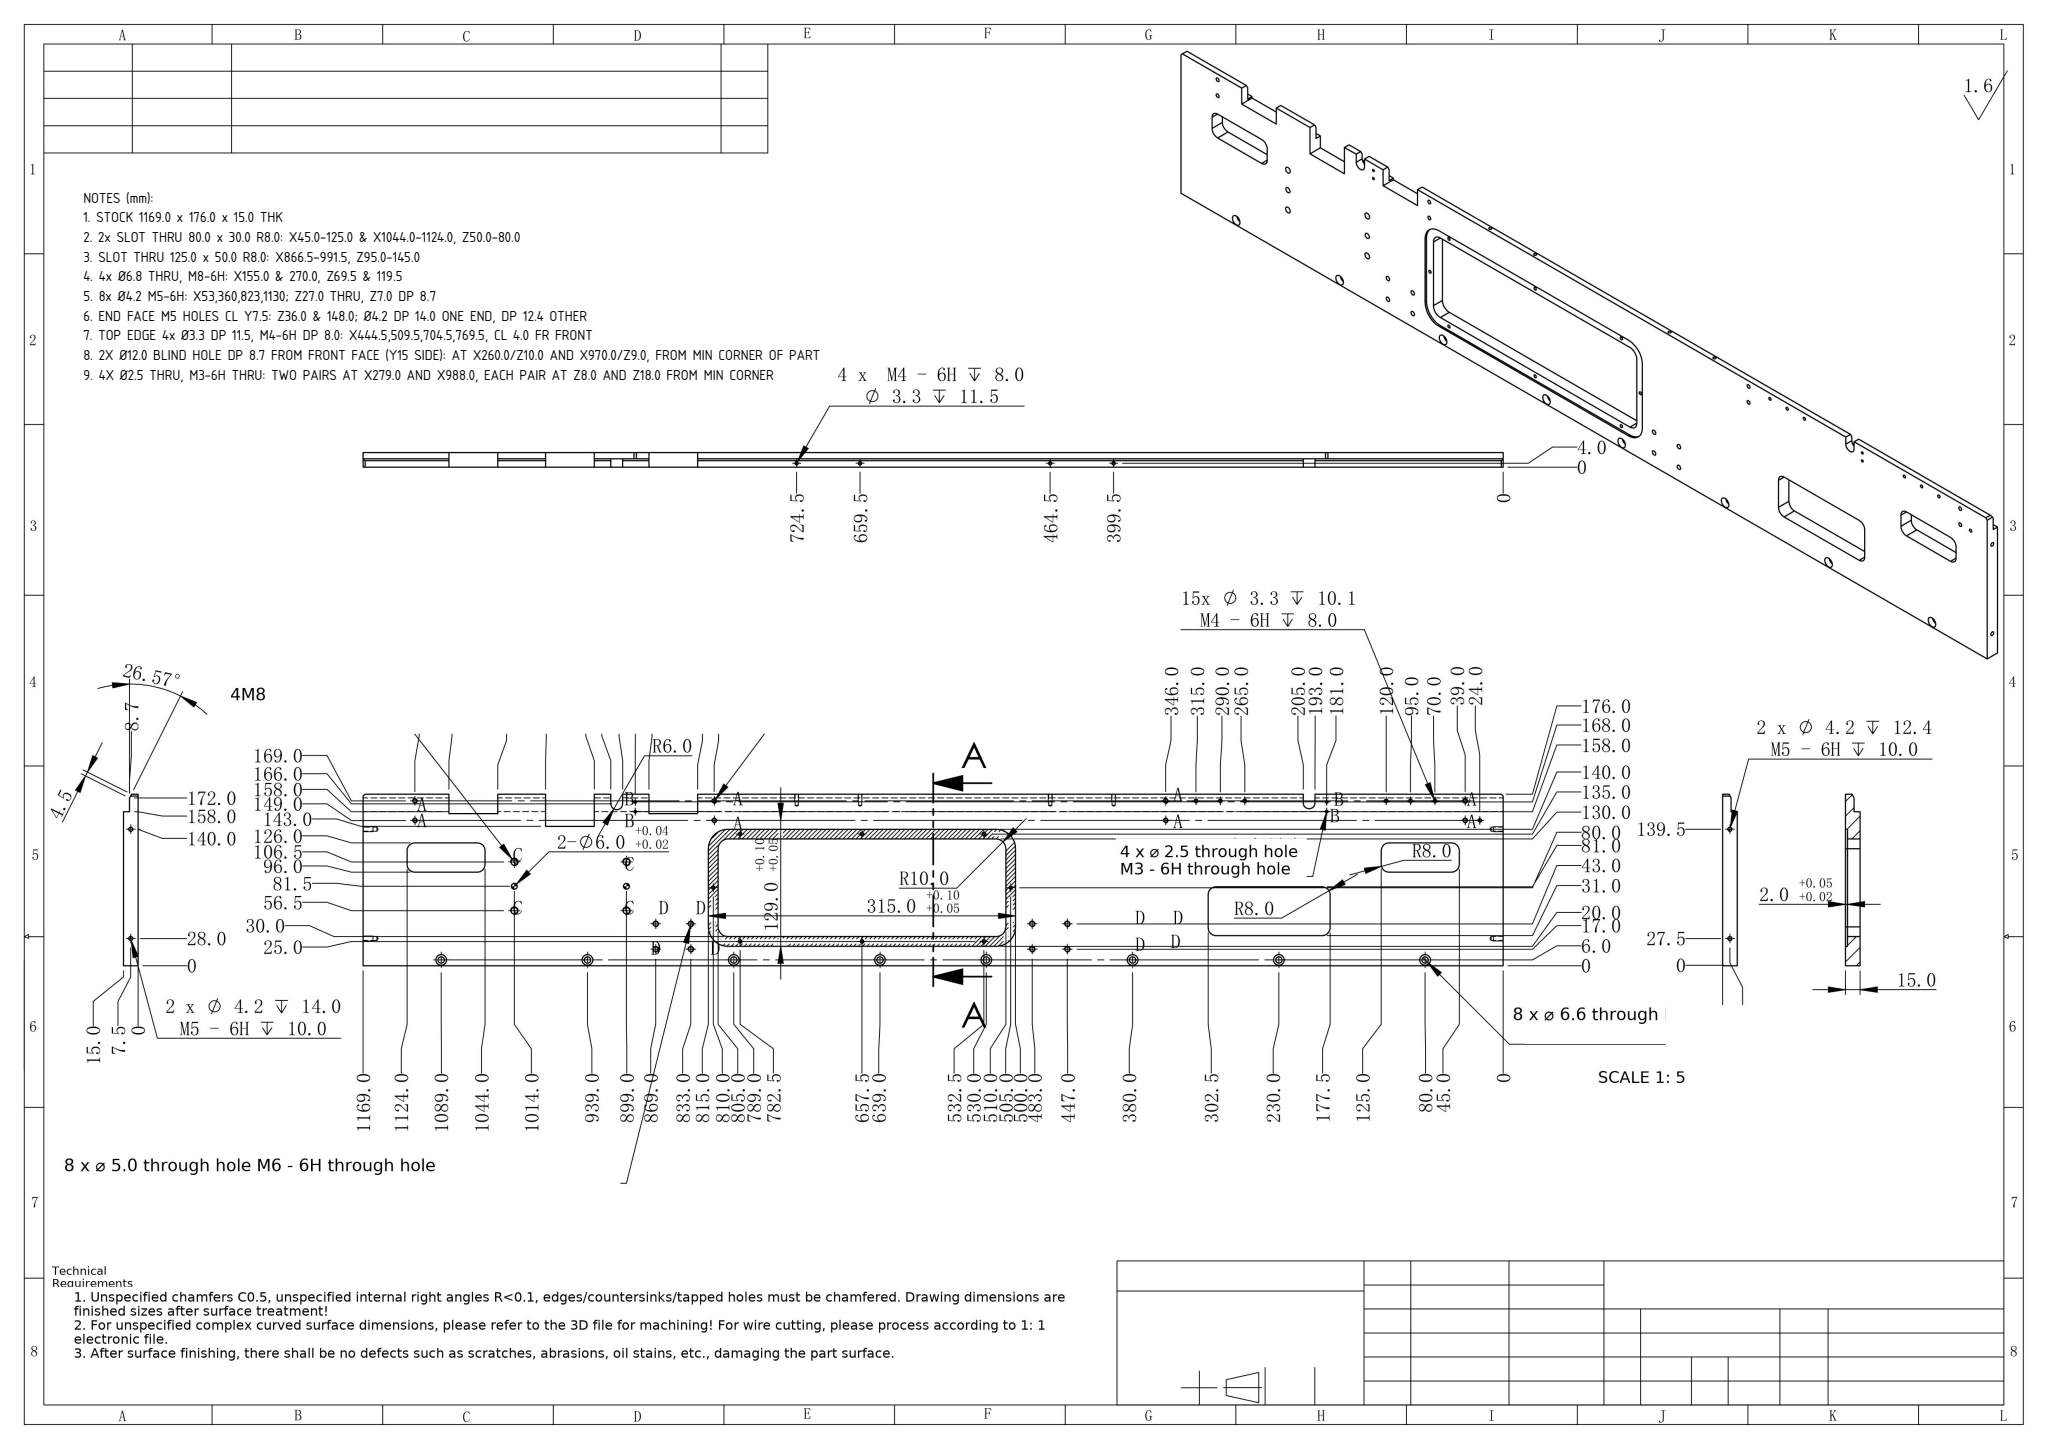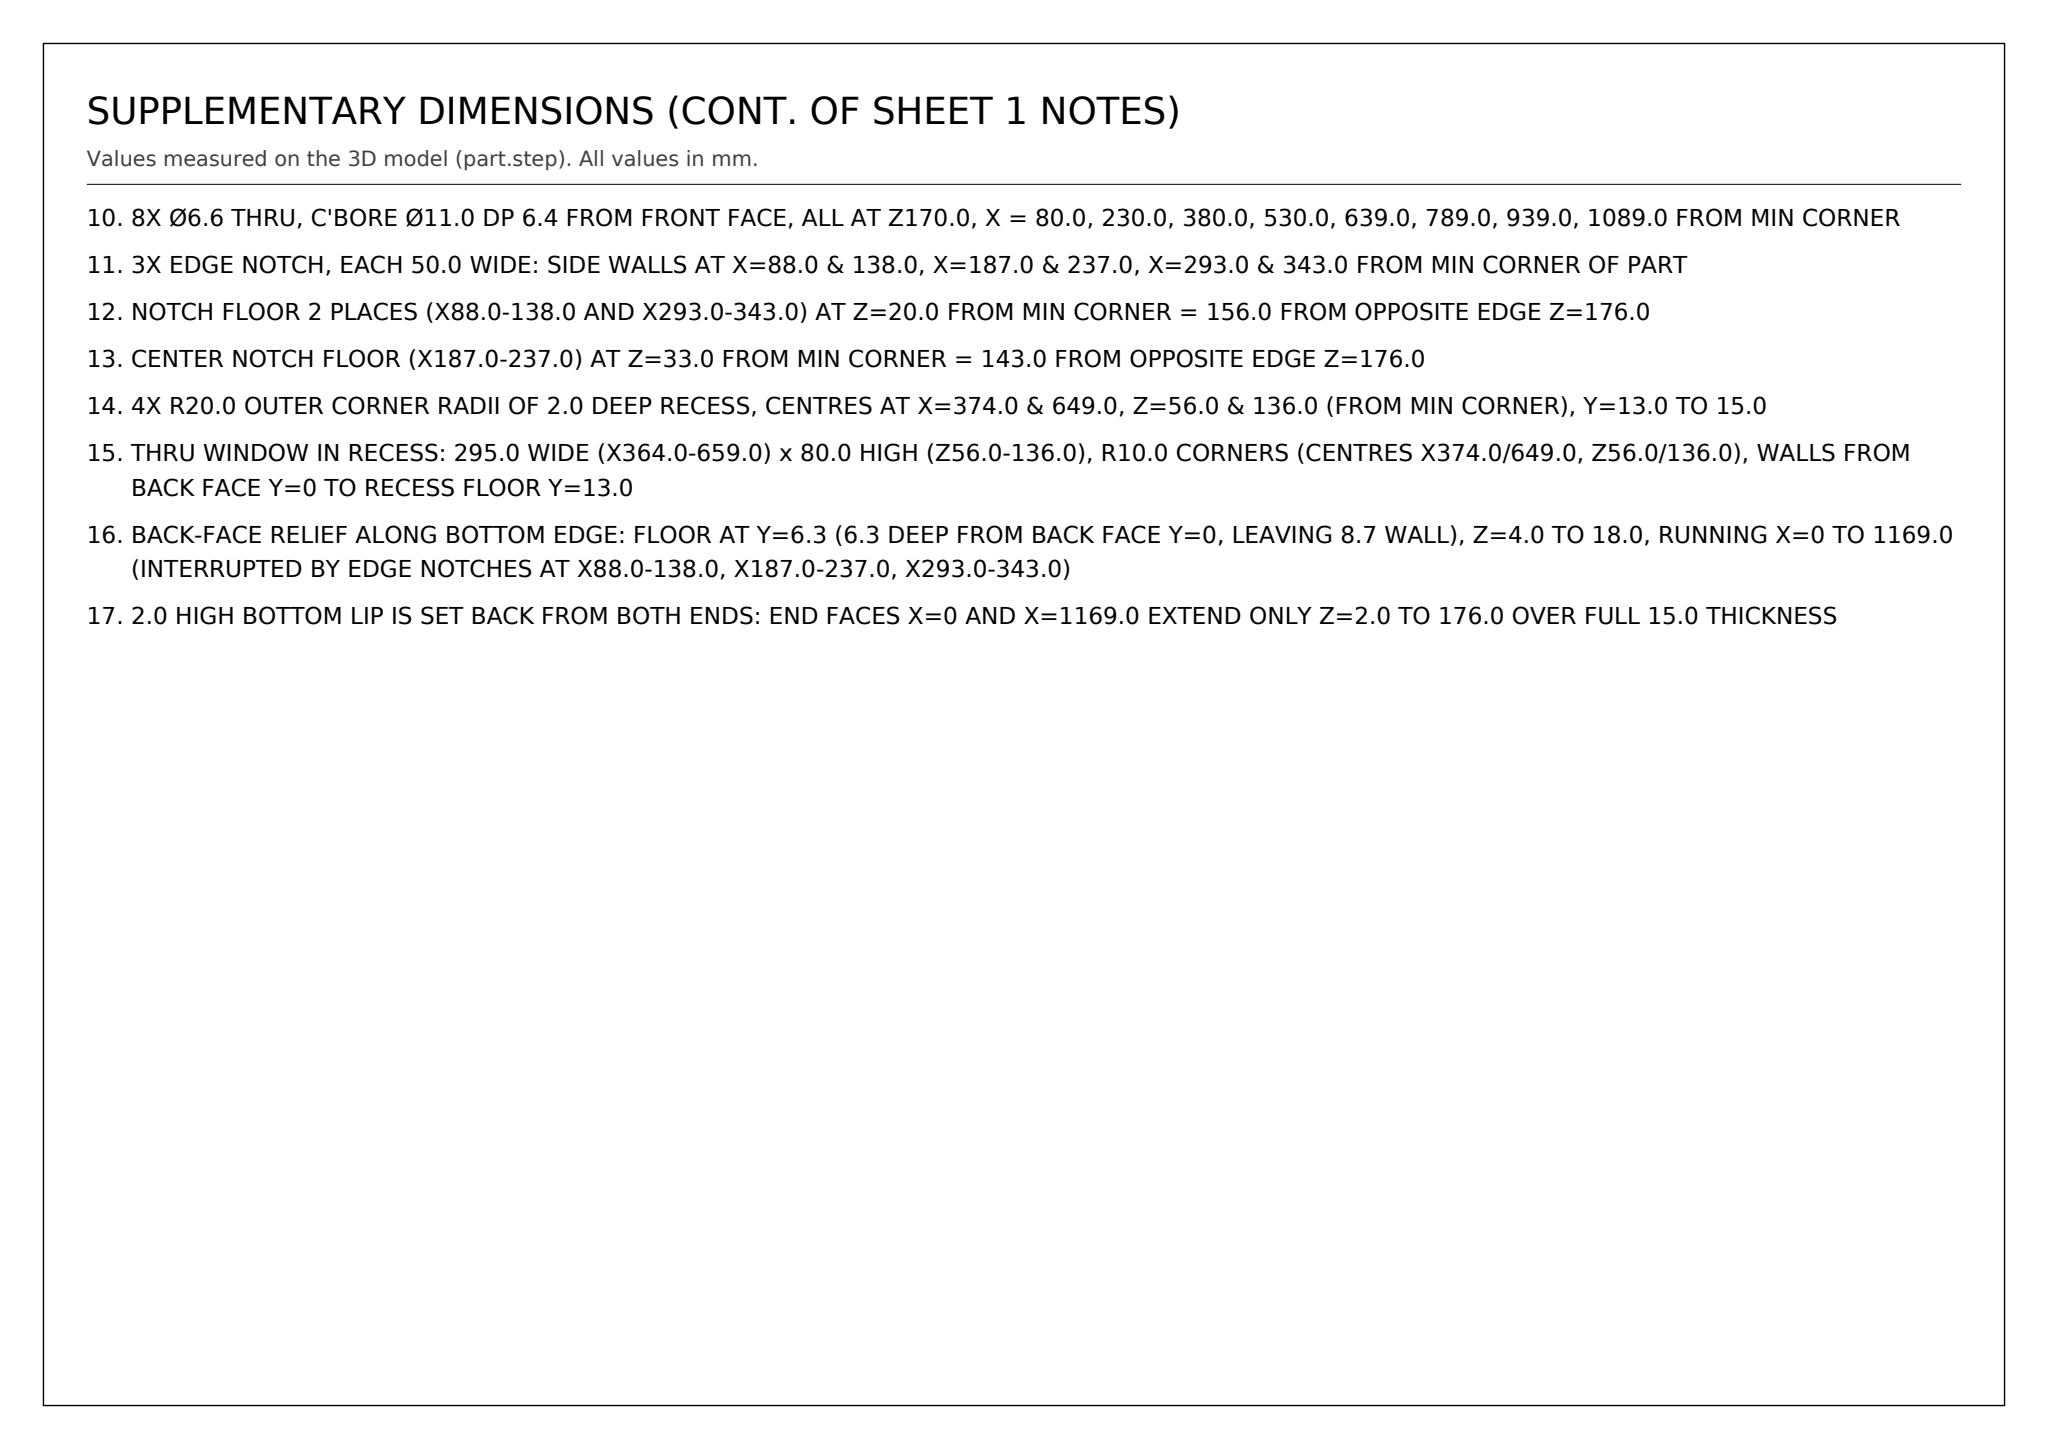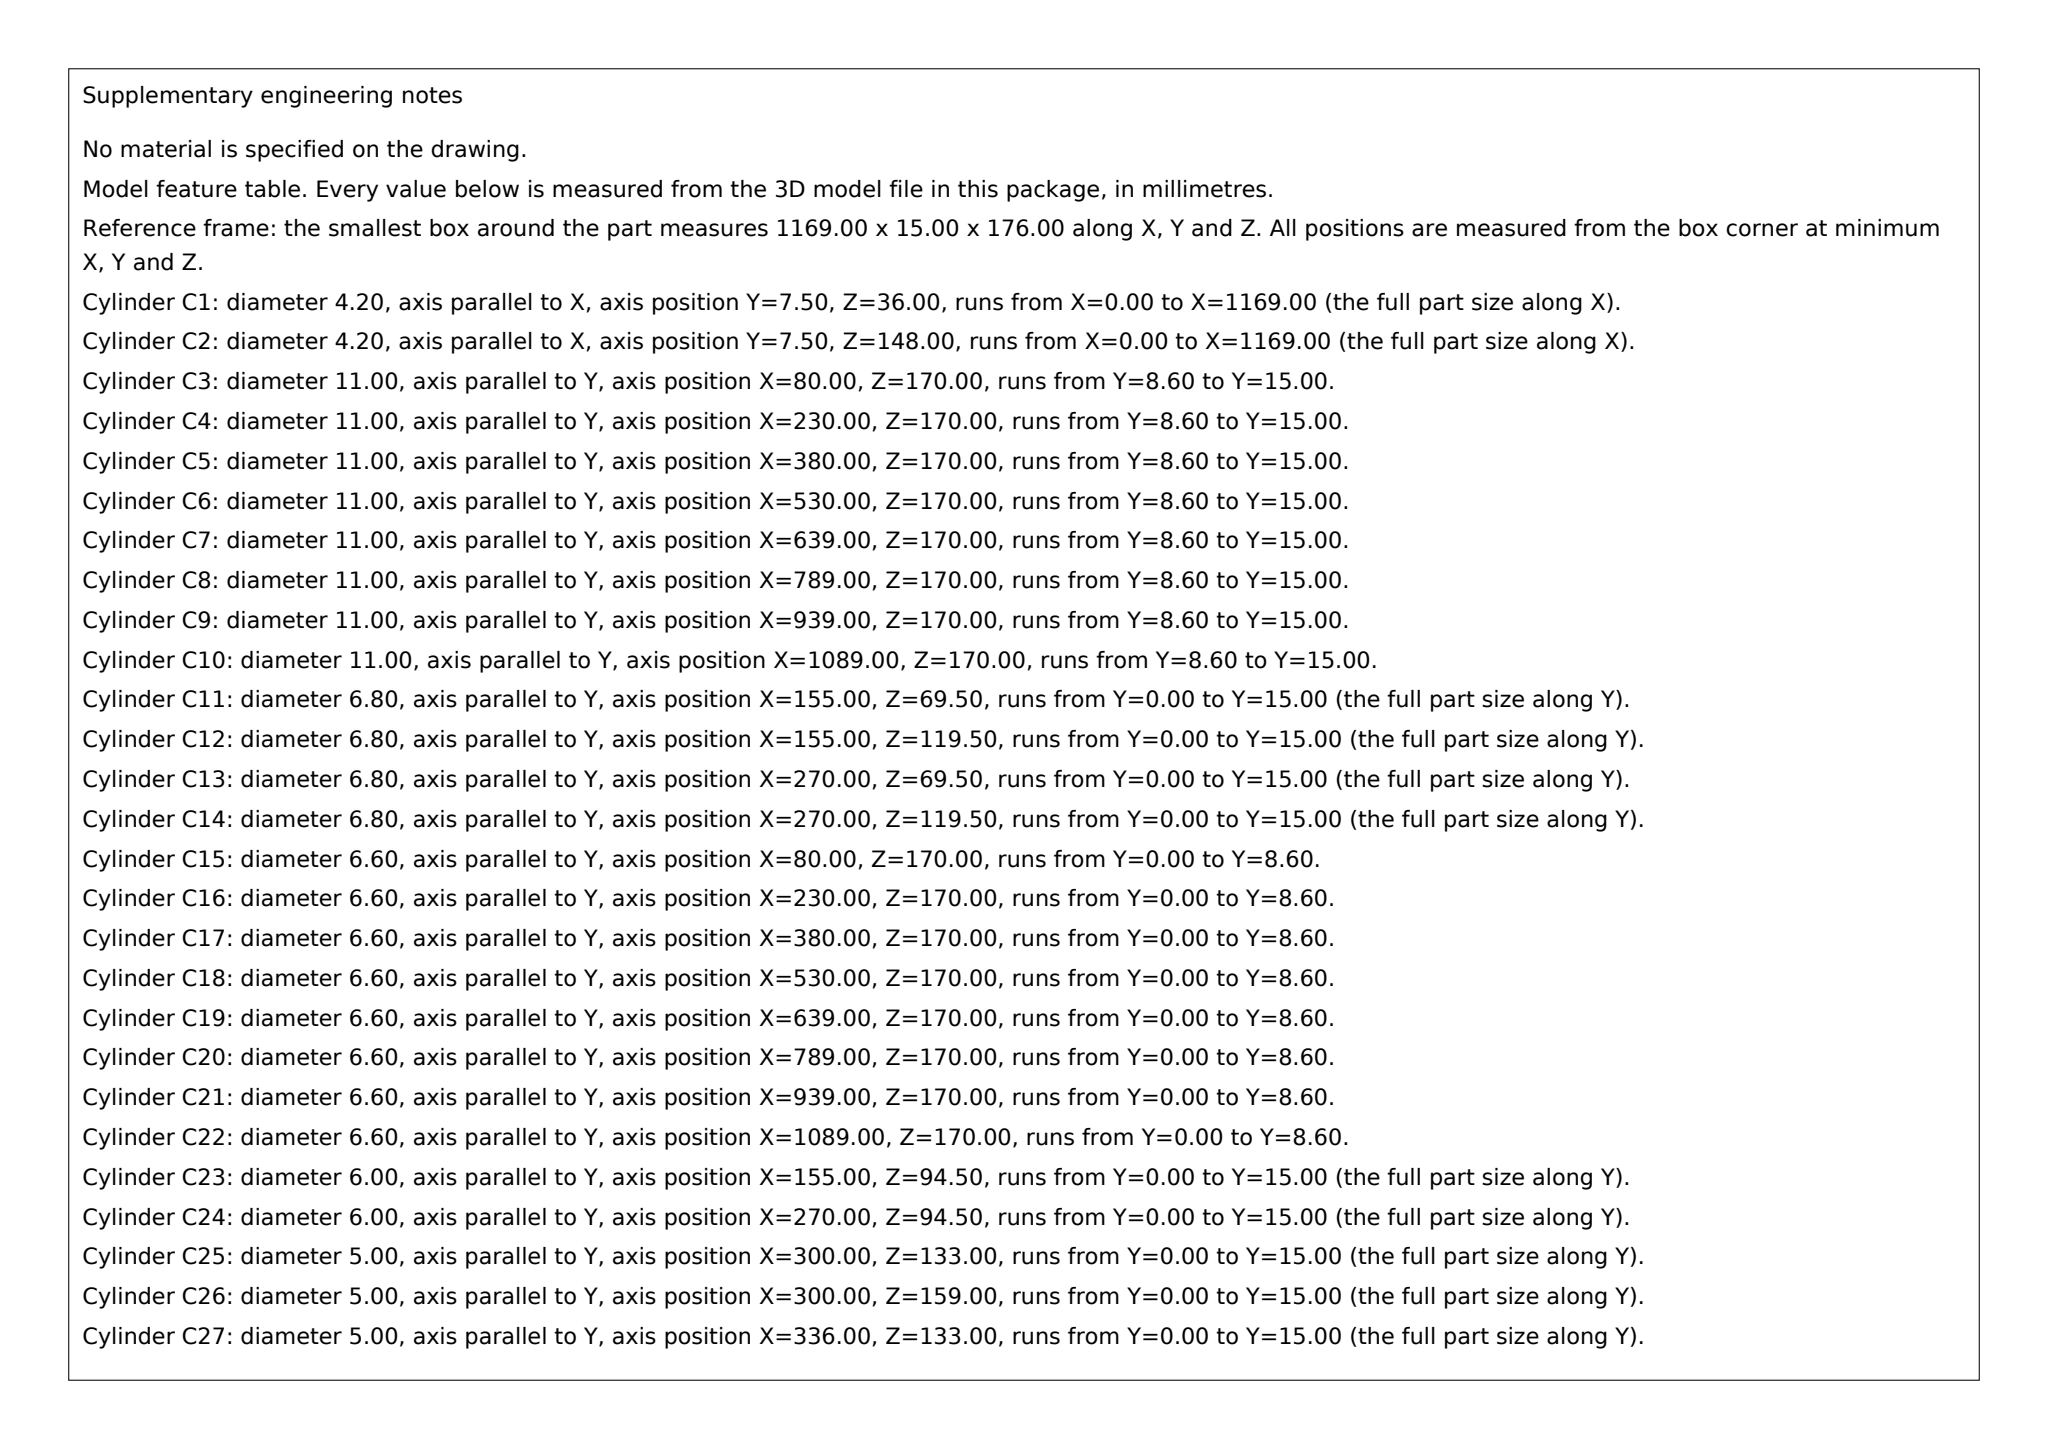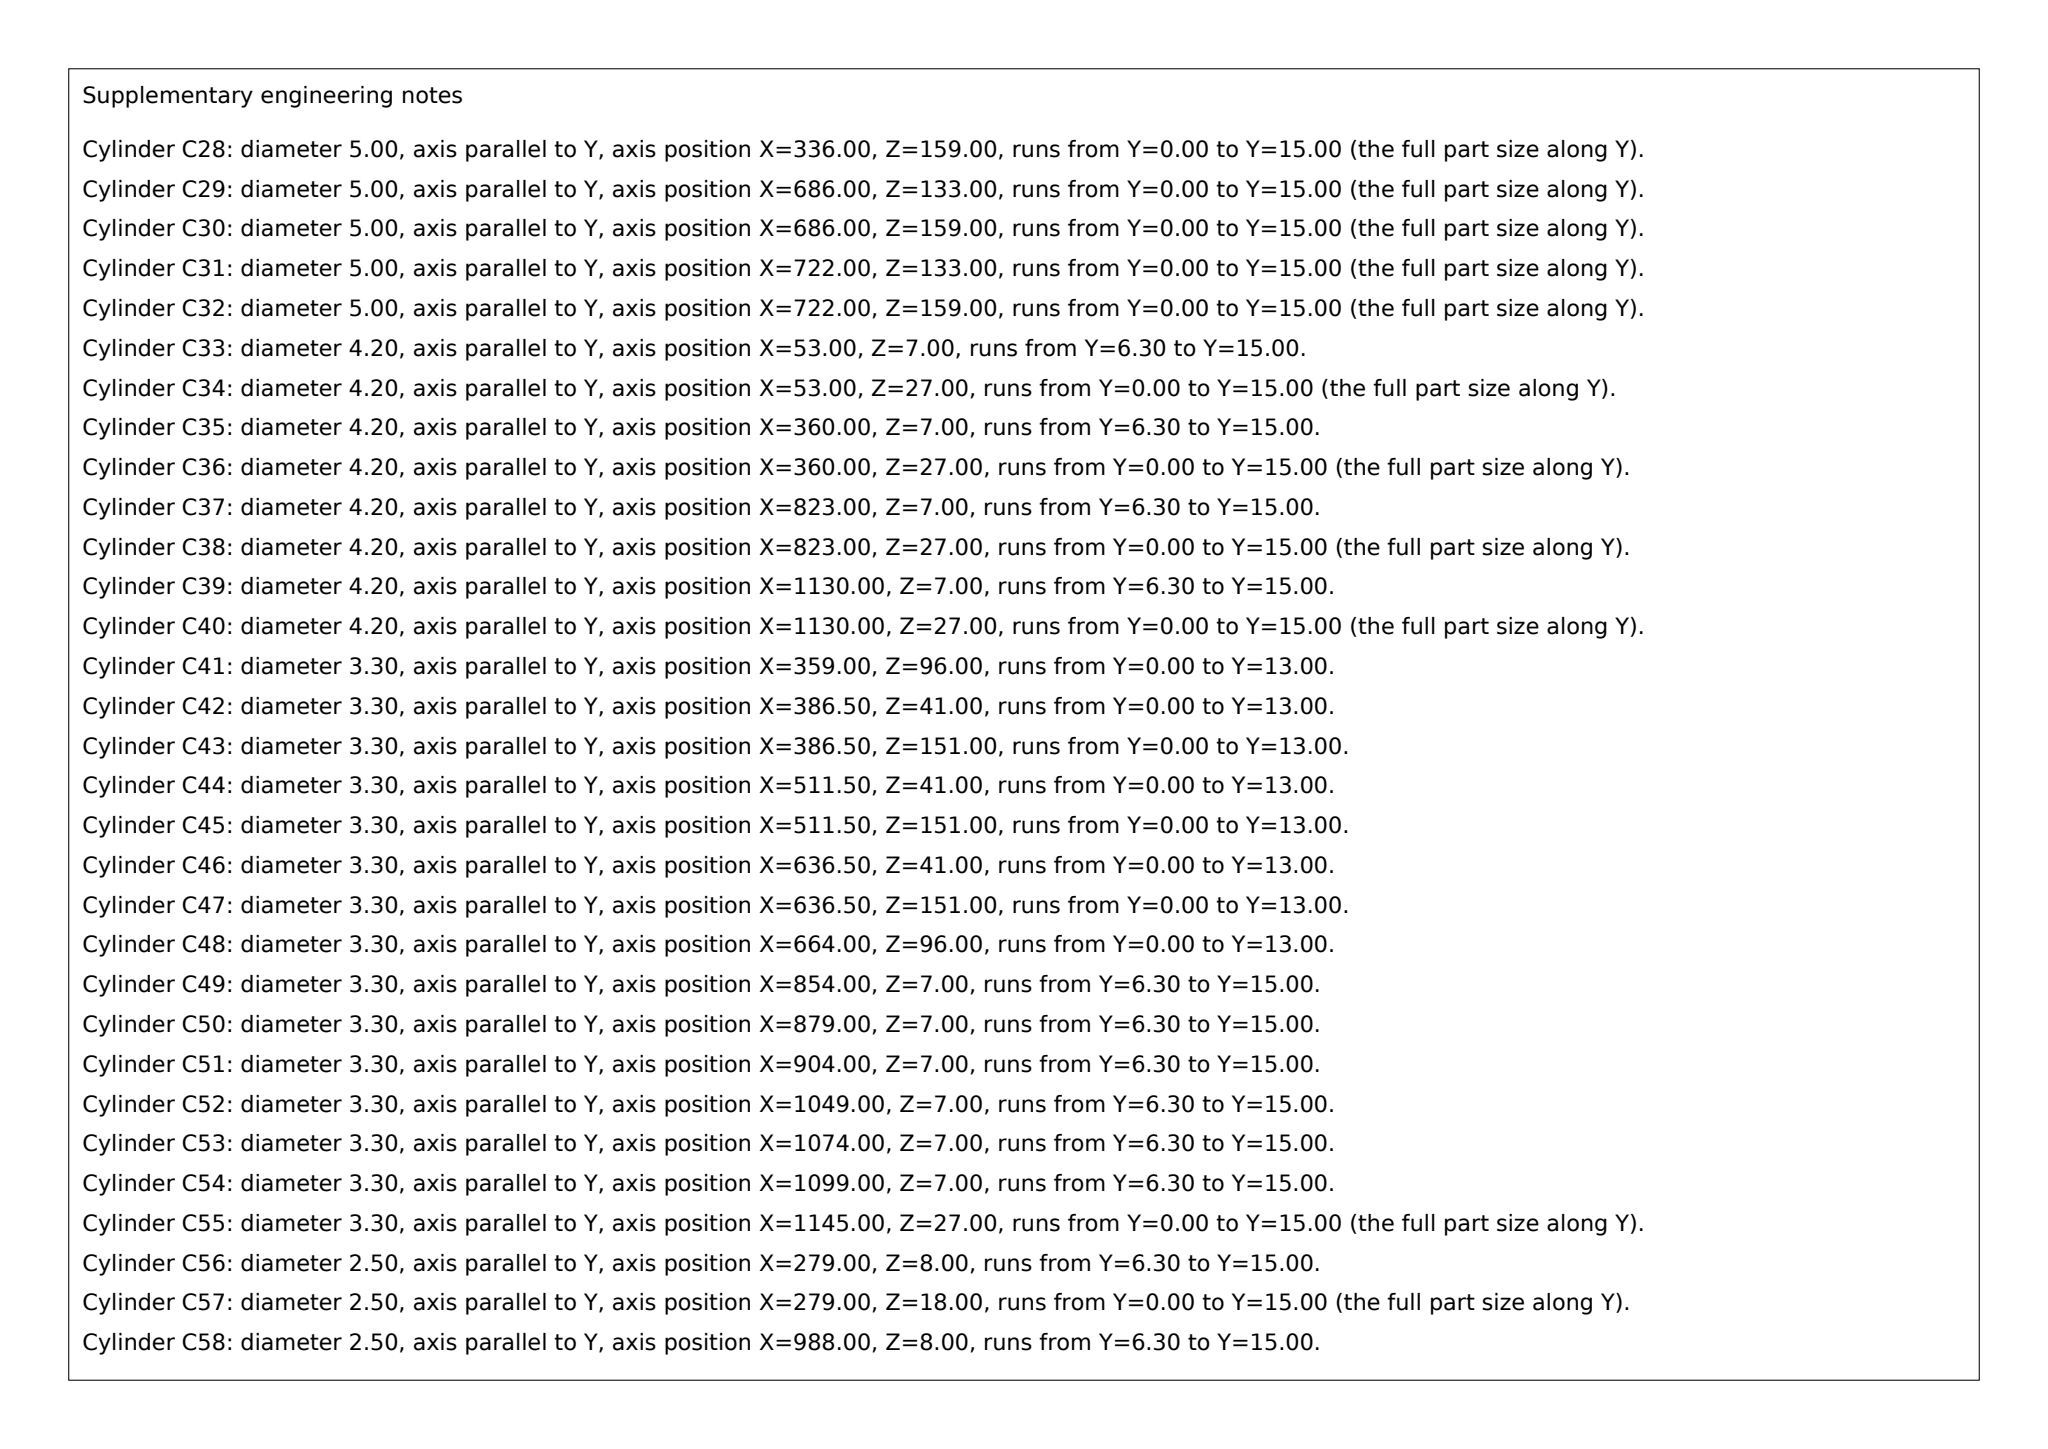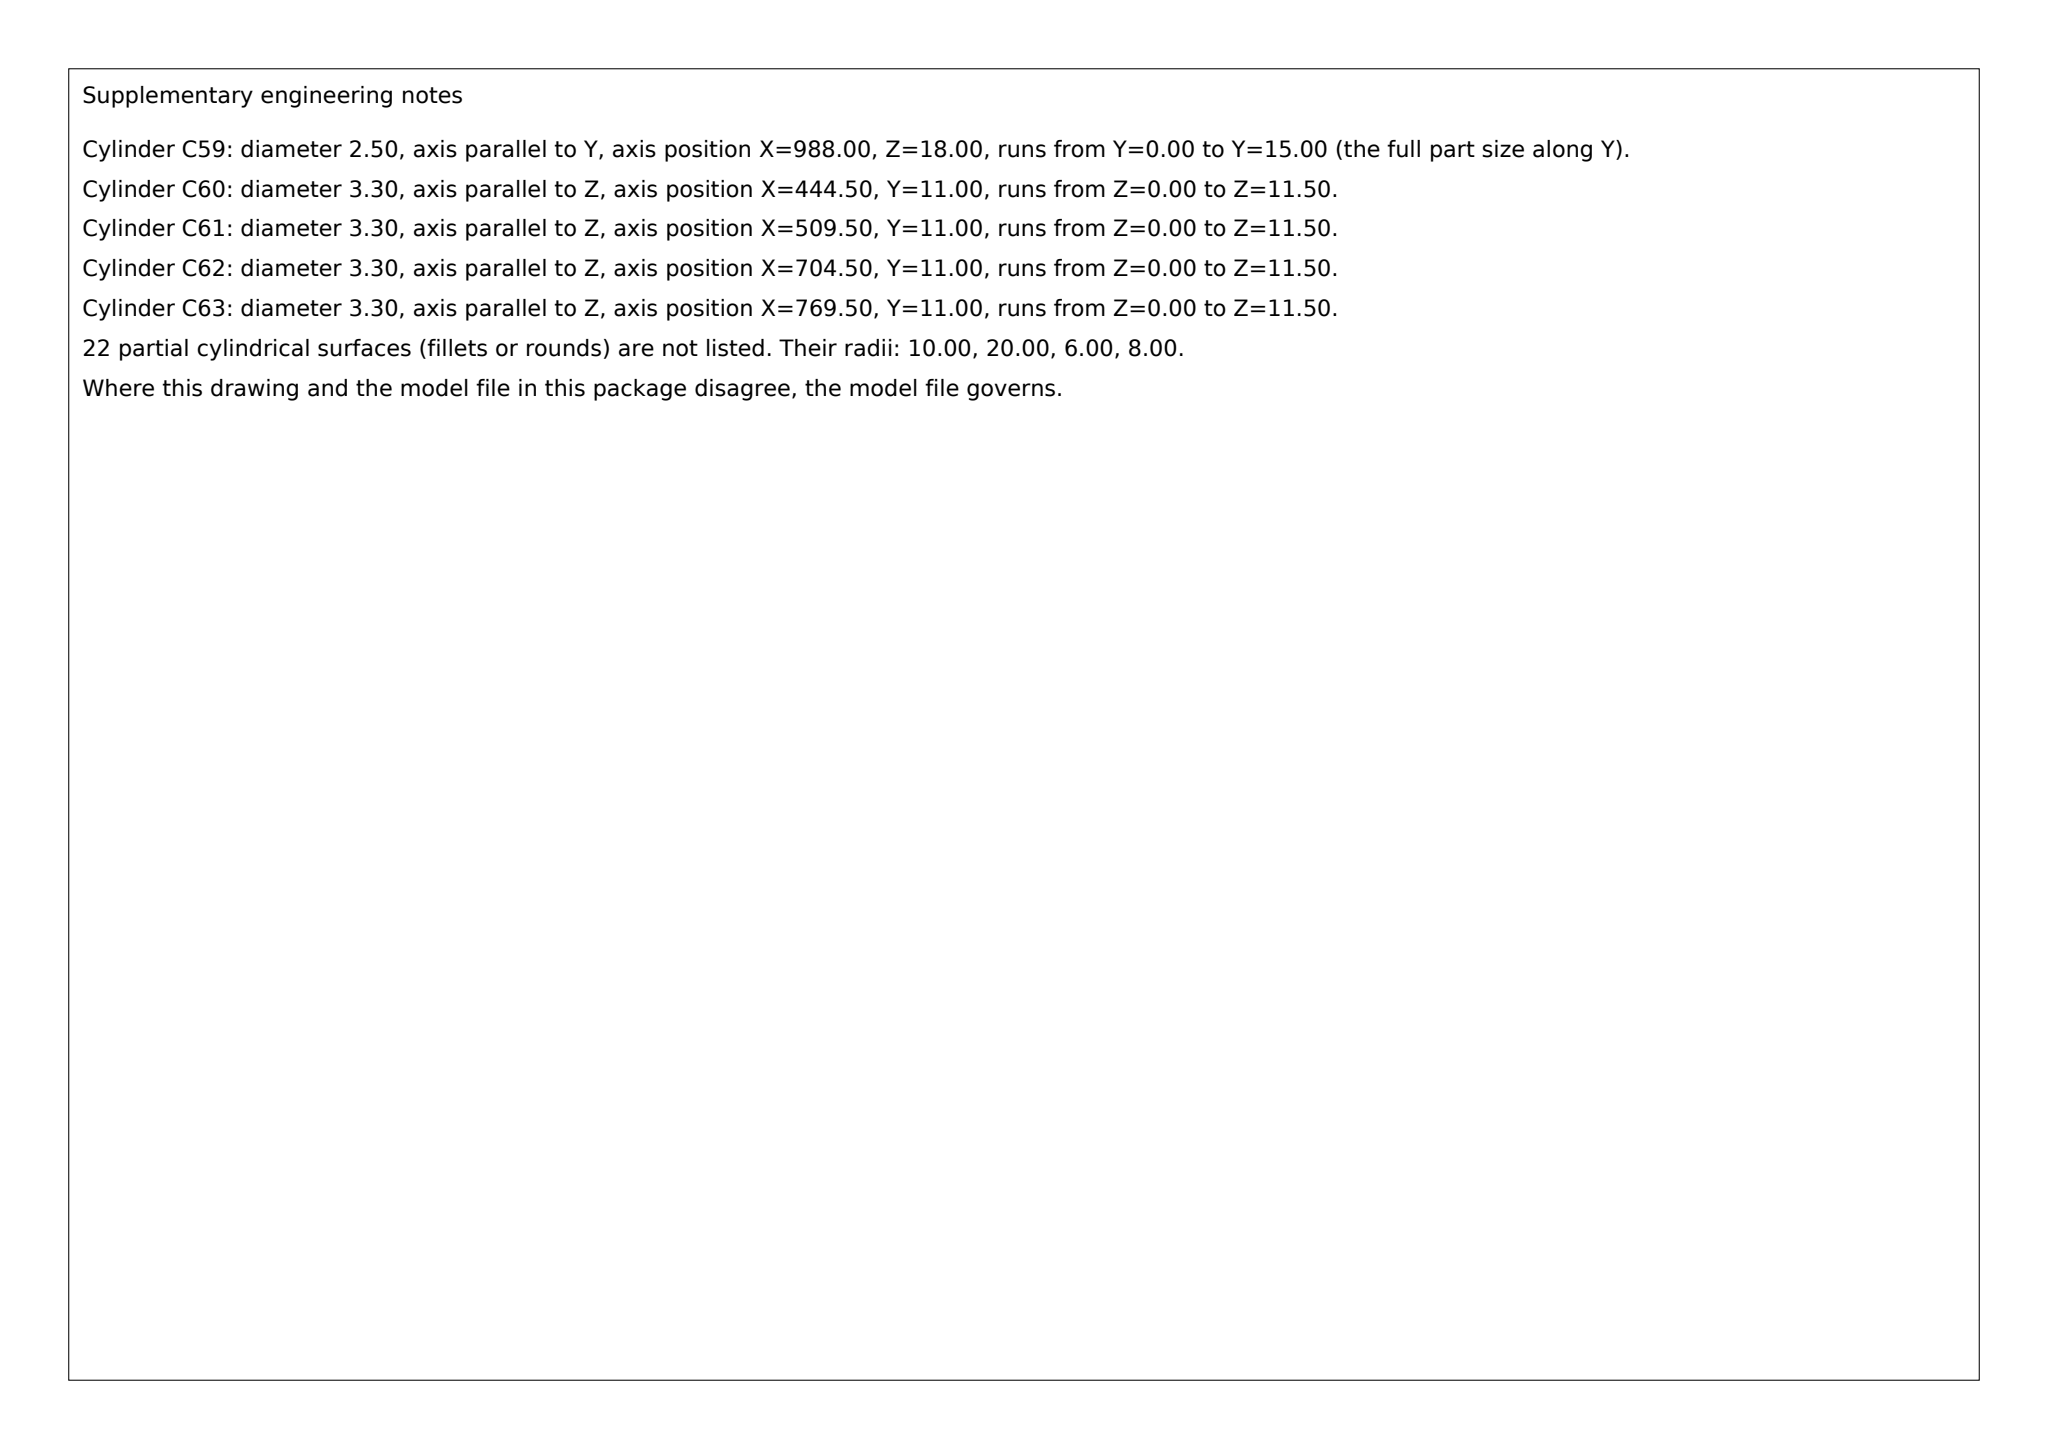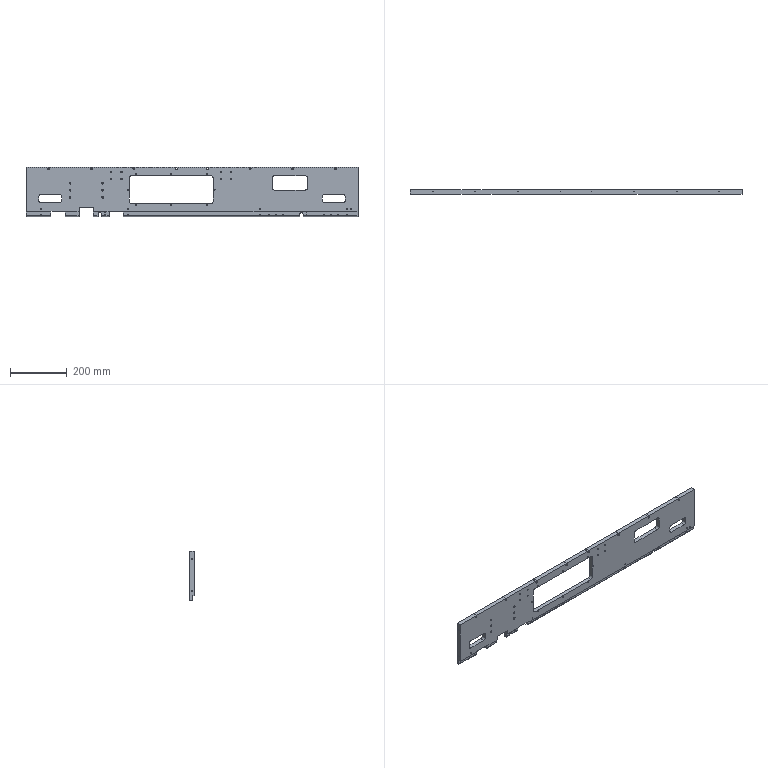Part | SolidWorks | mm | 1 solid | 239 faces | box 1169 x 15 x 176 mm | volume 2271563 mm3 | cylinder 152 | plane 71 | cone 16 | commonest cylinder face diameters 3.3 x38 4.2 x24 5 x16 11 x16 6.6 x16 16 x12 6.8 x8 2.5 x8
Drawing notes:
STOCK 1169.0 x 176.0 x 15.0 THK | from the solid: bbox_xyz [1169.0, 15.0, 176.0]
2x SLOT THRU 80.0 x 30.0 R8.0: X45.0-125.0 & X1044.0-1124.0, Z50.0-80.0 | from the solid: x planes 45,125,1044,1124; z planes 50,80; Ø16 thru cyls x=53/117 & 1052/1116, z=58/72
SLOT THRU 125.0 x 50.0 R8.0: X866.5-991.5, Z95.0-145.0 | from the solid: x planes 866.5,991.5; z planes 95,145; Ø16 thru cyls x=874.5/983.5, z=103/137
4x Ø6.8 THRU, M8-6H: X155.0 & 270.0, Z69.5 & 119.5 | from the solid: cyl Ø6.8 y-axis len 15.0 = full thk, x=155/270, z=69.5/119.5
8x Ø4.2 M5-6H: X53,360,823,1130; Z27.0 THRU, Z7.0 DP 8.7 | from the solid: cyl Ø4.2 y-axis len 15.0 at z=27.0 and len 8.7 at z=7.0, x=53/360/823/1130
END FACE M5 HOLES CL Y7.5: Z36.0 & 148.0; Ø4.2 DP 14.0 ONE END, DP 12.4 OTHER | from the solid: cyl Ø4.2 x-axis at y=7.5, z=36.0 & 148.0, lengths 14.0 and 12.4
TOP EDGE 4x Ø3.3 DP 11.5, M4-6H DP 8.0: X444.5,509.5,704.5,769.5, CL 4.0 FR FRONT | from the solid: cyl Ø3.3 z-axis at y=11.0 (front face y=15.0 -> 4.0), x=444.5/509.5/704.5/769.5, len 11.5
2X Ø12.0 BLIND HOLE DP 8.7 FROM FRONT FACE (Y15 SIDE): AT X260.0/Z10.0 AND X970.0/Z9.0, FROM MIN CORNER OF PART | from the solid: Ø12.0 y-axis arcs at (x260,z10) and (x970,z9) run from y=6.3 to y=15.0, i.e. 8.7 deep measured from the y=15.0 face; y=0 is the back face (y=0 plane x0-1169, z18-176) and y=15.0 is the front face.
4X Ø2.5 THRU, M3-6H THRU: TWO PAIRS AT X279.0 AND X988.0, EACH PAIR AT Z8.0 AND Z18.0 FROM MIN CORNER | from the solid: cylinders [2.5,'y',[279.0,null,8.0]], [2.5,'y',[279.0,null,18.0]], [2.5,'y',[988.0,null,8.0]], [2.5,'y',[988.0,null,18.0]]
8X Ø6.6 THRU, C'BORE Ø11.0 DP 6.4 FROM FRONT FACE, ALL AT Z170.0, X = 80.0, 230.0, 380.0, 530.0, 639.0, 789.0, 939.0, 1089.0 FROM MIN CORNER | from the solid: Ø11.0 bores at z=170.0 (x=80,230,380,530,639,789,939,1089) run y=8.6 to y=15.0 = 6.4 deep from the y=15.0 front face; y=8.6 planes are the c'bore floors.
3X EDGE NOTCH, EACH 50.0 WIDE: SIDE WALLS AT X=88.0 & 138.0, X=187.0 & 237.0, X=293.0 & 343.0 FROM MIN CORNER OF PART | from the solid: axis_planes normal x at offsets 88.0, 138.0, 187.0, 237.0, 293.0, 343.0 (y extent 0-15, full thickness notch walls)
NOTCH FLOOR 2 PLACES (X88.0-138.0 AND X293.0-343.0) AT Z=20.0 FROM MIN CORNER = 156.0 FROM OPPOSITE EDGE Z=176.0 | from the solid: axis_planes x=88.0, 138.0, 293.0, 343.0 each with z extent [0.0, 20.0]; bbox_xyz z = 176.0
CENTER NOTCH FLOOR (X187.0-237.0) AT Z=33.0 FROM MIN CORNER = 143.0 FROM OPPOSITE EDGE Z=176.0 | from the solid: axis_planes x=187.0 and x=237.0 each with z extent [0.0, 33.0]; bbox_xyz z = 176.0
4X R20.0 OUTER CORNER RADII OF 2.0 DEEP RECESS, CENTRES AT X=374.0 & 649.0, Z=56.0 & 136.0 (FROM MIN CORNER), Y=13.0 TO 15.0 | from the solid: cylinders: 4X concave arc dia 40.0, axis y, at (374.0,Z56.0), (374.0,Z136.0), (649.0,Z56.0), (649.0,Z136.0), from y13.0 to y15.0, 90 deg
THRU WINDOW IN RECESS: 295.0 WIDE (X364.0-659.0) x 80.0 HIGH (Z56.0-136.0), R10.0 CORNERS (CENTRES X374.0/649.0, Z56.0/136.0), WALLS FROM BACK FACE Y=0 TO RECESS FLOOR Y=13.0 | from the solid: axis_planes normal x at 364.0 and 659.0, extent y[0.0,13.0] z[56.0,136.0]; 4X concave arc dia 20.0 axis y at X374.0/649.0, Z56.0/136.0, from y0.0 to y13.0
BACK-FACE RELIEF ALONG BOTTOM EDGE: FLOOR AT Y=6.3 (6.3 DEEP FROM BACK FACE Y=0, LEAVING 8.7 WALL), Z=4.0 TO 18.0, RUNNING X=0 TO 1169.0 (INTERRUPTED BY EDGE NOTCHES AT X88.0-138.0, X187.0-237.0, X293.0-343.0) | from the solid: axis_planes normal y, offset 6.3, extents x[0.0,88.0], x[138.0,187.0], x[237.0,293.0], x[343.0,1169.0], all z[4.0,18.0]; back face plane y=0.0 extent z[18.0,176.0]
2.0 HIGH BOTTOM LIP IS SET BACK FROM BOTH ENDS: END FACES X=0 AND X=1169.0 EXTEND ONLY Z=2.0 TO 176.0 OVER FULL 15.0 THICKNESS | from the solid: axis_planes normal x, offsets 0.0 and 1169.0, extent y[0.0,15.0] z[2.0,176.0]